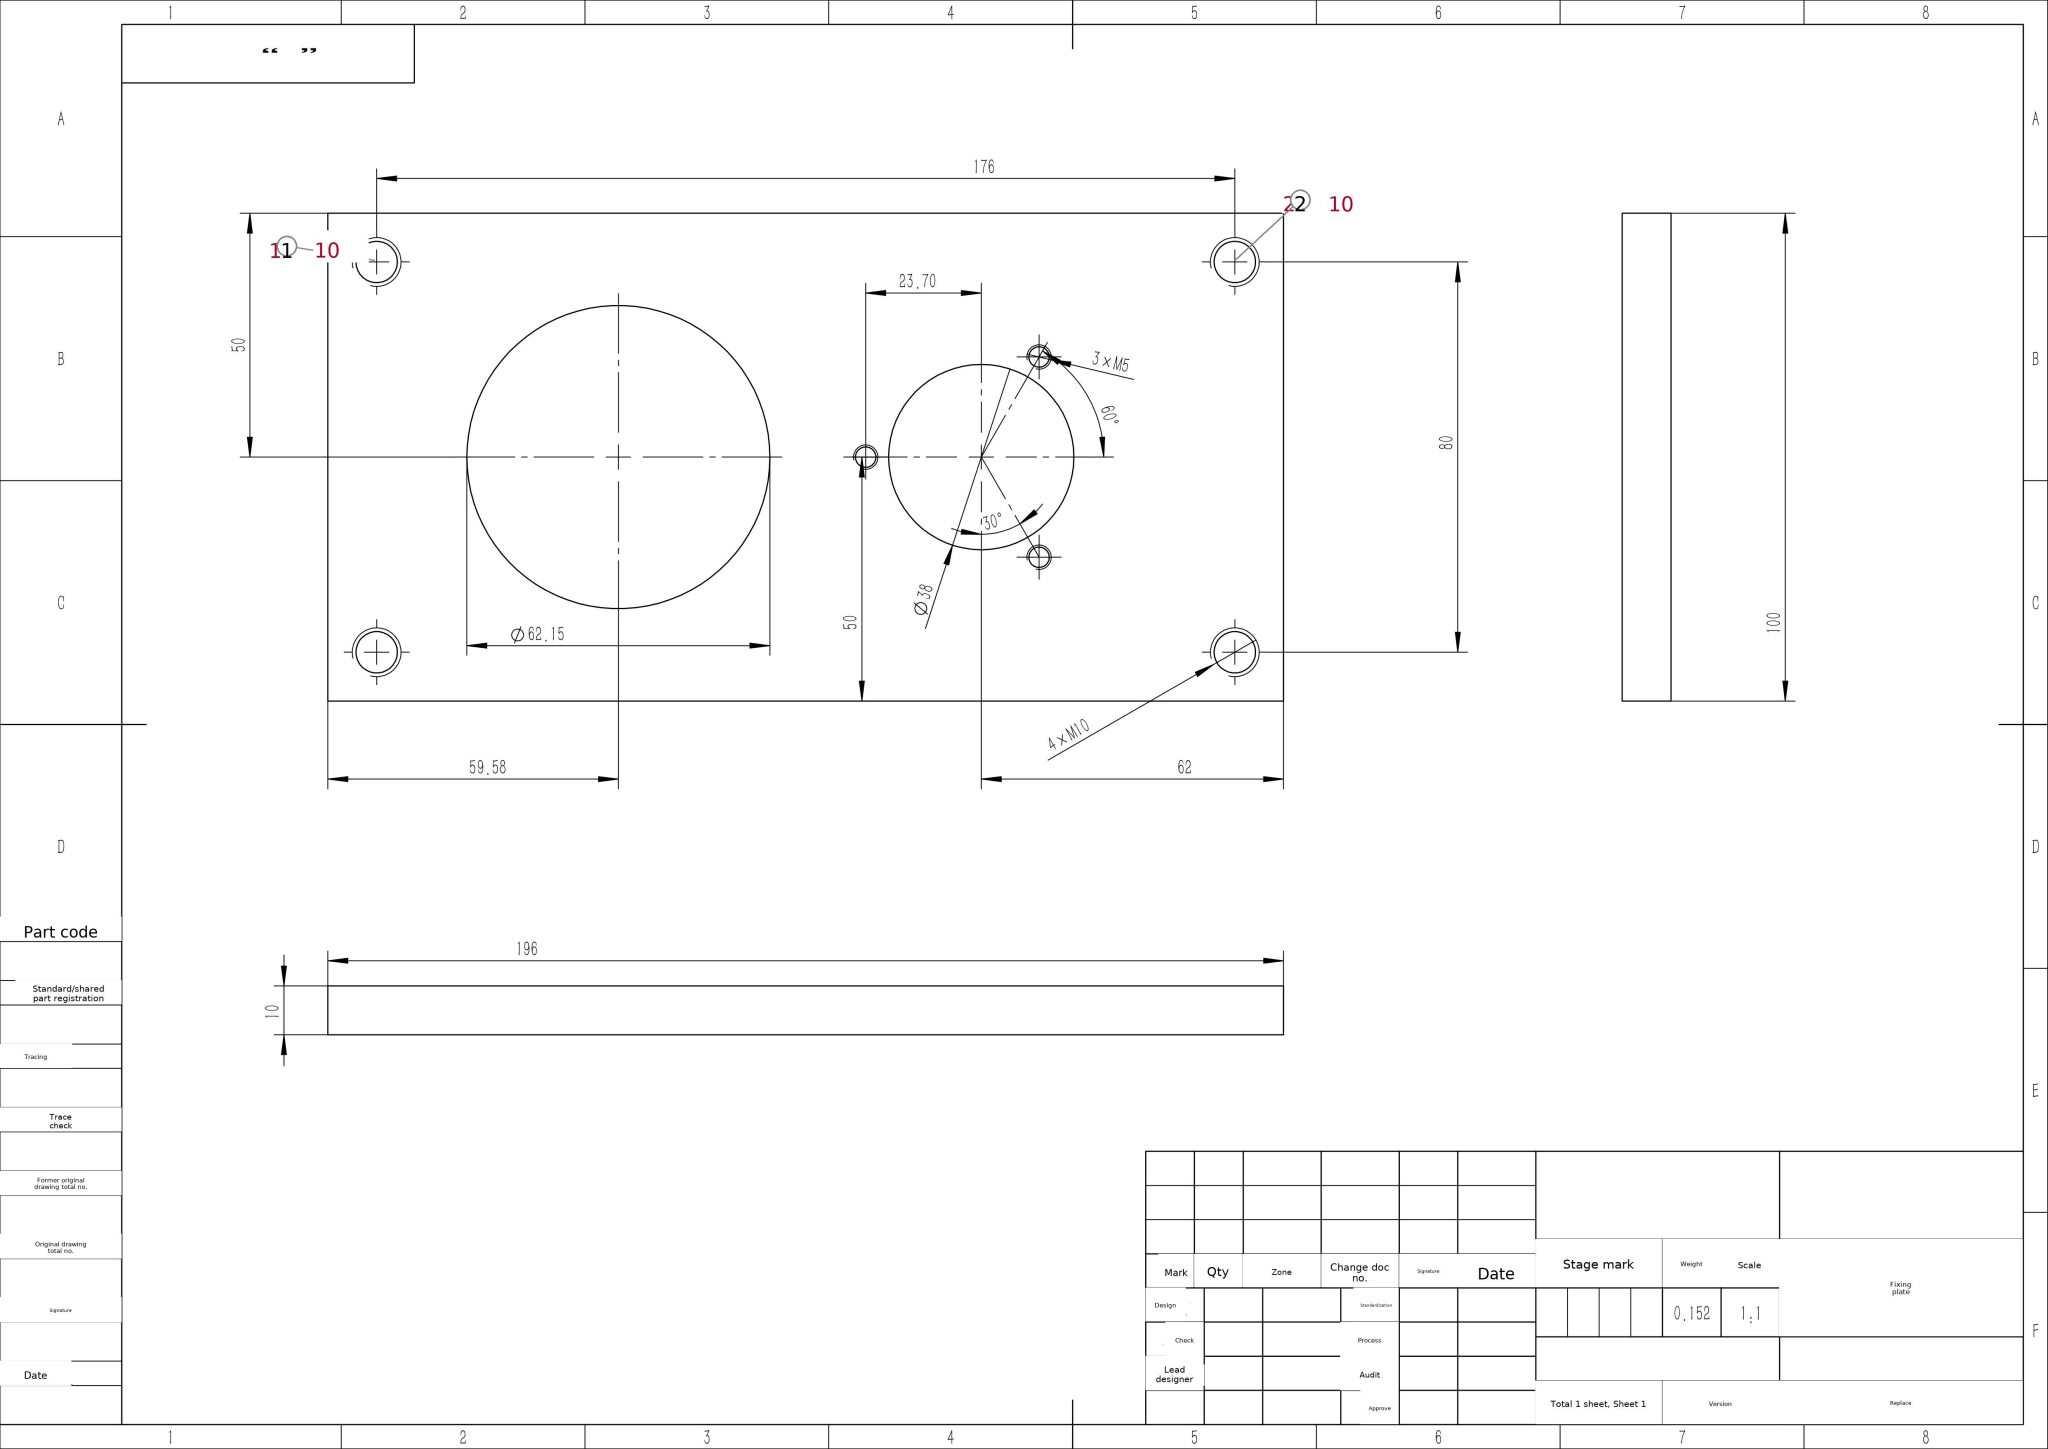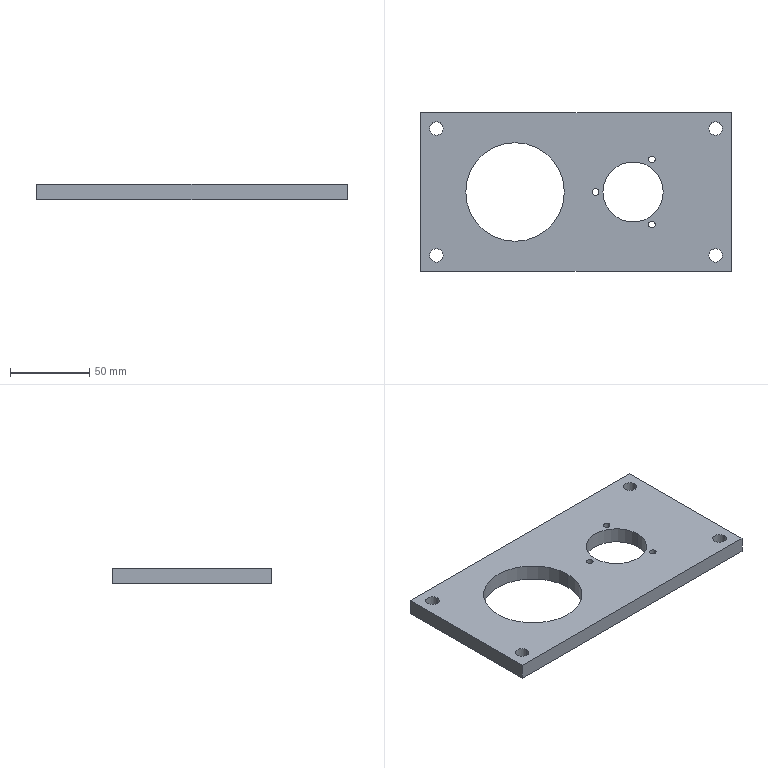Part | SolidWorks | mm | 1 solid | 24 faces | box 196 x 100 x 10 mm | volume 151636 mm3 | cylinder 18 | plane 6 | commonest cylinder face diameters 8.5 x8 4.2 x6 62.15 x2 38 x2
build123d program:
from build123d import *

# Parameters (mm, degrees)
SKETCH1_W           = 196
SKETCH1_H           = 100
BOSS_EXTRUDE1_DEPTH = 10
SKETCH2_R           = 31.075
SKETCH2_R_2         = 19
CUT_EXTRUDE1_DEPTH  = 10
M10_TAPPED_HOLE1_D  = 8.5
M5_TAPPED_HOLE1_D   = 4.2


with BuildPart() as part:
    # Sketch1 → Boss-Extrude1 (new body)
    with BuildSketch(Plane.XY):
        Rectangle(SKETCH1_W, SKETCH1_H)
    extrude(amount=BOSS_EXTRUDE1_DEPTH)

    # Sketch2 → Cut-Extrude1 (cut)
    with BuildSketch(Plane.XY):
        with Locations((-38.425, 0)):
            Circle(SKETCH2_R)
        with Locations((36, 0)):
            Circle(SKETCH2_R_2)
    extrude(amount=CUT_EXTRUDE1_DEPTH, mode=Mode.SUBTRACT)

    # M10 Tapped Hole1 (through all)
    with Locations(Plane.XY.offset(10)):
        with Locations((88, 40), (88, -40), (-88, -40), (-88, 40)):
            Hole(M10_TAPPED_HOLE1_D / 2)

    # M5 Tapped Hole1 (through all)
    with Locations(Plane.XY.offset(10)):
        with Locations((47.85, 20.525), (12.3, 0), (47.85, -20.525)):
            Hole(M5_TAPPED_HOLE1_D / 2)


solid = part.part
STEP:
#1=CARTESIAN_POINT('',(45.75,20.525,0.));
#2=VERTEX_POINT('',#1);
#3=CARTESIAN_POINT('',(49.95,20.525,0.));
#4=VERTEX_POINT('',#3);
#5=CARTESIAN_POINT('',(47.85,20.525,0.));
#6=DIRECTION('',(0.,0.,1.));
#7=DIRECTION('',(1.,0.,0.));
#8=AXIS2_PLACEMENT_3D('',#5,#6,#7);
#9=CIRCLE('',#8,2.1);
#10=EDGE_CURVE('',#2,#4,#9,.T.);
#11=ORIENTED_EDGE('',*,*,#10,.F.);
#12=CARTESIAN_POINT('',(45.75,20.525,10.));
#13=VERTEX_POINT('',#12);
#14=CARTESIAN_POINT('',(45.75,20.525,10.));
#15=DIRECTION('',(0.,0.,1.));
#16=VECTOR('',#15,1000.);
#17=LINE('',#14,#16);
#18=EDGE_CURVE('',#2,#13,#17,.T.);
#19=ORIENTED_EDGE('',*,*,#18,.T.);
#20=CARTESIAN_POINT('',(49.95,20.525,10.));
#21=VERTEX_POINT('',#20);
#22=CARTESIAN_POINT('',(47.85,20.525,10.));
#23=DIRECTION('',(0.,0.,1.));
#24=DIRECTION('',(1.,0.,0.));
#25=AXIS2_PLACEMENT_3D('',#22,#23,#24);
#26=CIRCLE('',#25,2.1);
#27=EDGE_CURVE('',#13,#21,#26,.T.);
#28=ORIENTED_EDGE('',*,*,#27,.T.);
#29=CARTESIAN_POINT('',(49.95,20.525,10.));
#30=DIRECTION('',(0.,0.,1.));
#31=VECTOR('',#30,1000.);
#32=LINE('',#29,#31);
#33=EDGE_CURVE('',#4,#21,#32,.T.);
#34=ORIENTED_EDGE('',*,*,#33,.F.);
#35=EDGE_LOOP('',(#11,#19,#28,#34));
#36=FACE_OUTER_BOUND('',#35,.T.);
#37=CARTESIAN_POINT('',(47.85,20.525,10.));
#38=DIRECTION('',(0.,0.,1.));
#39=DIRECTION('',(1.,0.,0.));
#40=AXIS2_PLACEMENT_3D('',#37,#38,#39);
#41=CYLINDRICAL_SURFACE('',#40,2.1);
#42=ADVANCED_FACE('',(#36),#41,.F.);
#43=CARTESIAN_POINT('',(10.2,-0.,0.));
#44=VERTEX_POINT('',#43);
#45=CARTESIAN_POINT('',(14.4,-0.,0.));
#46=VERTEX_POINT('',#45);
#47=CARTESIAN_POINT('',(12.3,-0.,0.));
#48=DIRECTION('',(0.,0.,1.));
#49=DIRECTION('',(1.,0.,0.));
#50=AXIS2_PLACEMENT_3D('',#47,#48,#49);
#51=CIRCLE('',#50,2.1);
#52=EDGE_CURVE('',#44,#46,#51,.T.);
#53=ORIENTED_EDGE('',*,*,#52,.F.);
#54=CARTESIAN_POINT('',(10.2,-0.,10.));
#55=VERTEX_POINT('',#54);
#56=CARTESIAN_POINT('',(10.2,-0.,10.));
#57=DIRECTION('',(0.,0.,1.));
#58=VECTOR('',#57,1000.);
#59=LINE('',#56,#58);
#60=EDGE_CURVE('',#44,#55,#59,.T.);
#61=ORIENTED_EDGE('',*,*,#60,.T.);
#62=CARTESIAN_POINT('',(14.4,-0.,10.));
#63=VERTEX_POINT('',#62);
#64=CARTESIAN_POINT('',(12.3,-0.,10.));
#65=DIRECTION('',(0.,0.,1.));
#66=DIRECTION('',(1.,0.,0.));
#67=AXIS2_PLACEMENT_3D('',#64,#65,#66);
#68=CIRCLE('',#67,2.1);
#69=EDGE_CURVE('',#55,#63,#68,.T.);
#70=ORIENTED_EDGE('',*,*,#69,.T.);
#71=CARTESIAN_POINT('',(14.4,-0.,10.));
#72=DIRECTION('',(0.,0.,1.));
#73=VECTOR('',#72,1000.);
#74=LINE('',#71,#73);
#75=EDGE_CURVE('',#46,#63,#74,.T.);
#76=ORIENTED_EDGE('',*,*,#75,.F.);
#77=EDGE_LOOP('',(#53,#61,#70,#76));
#78=FACE_OUTER_BOUND('',#77,.T.);
#79=CARTESIAN_POINT('',(12.3,-0.,10.));
#80=DIRECTION('',(0.,0.,1.));
#81=DIRECTION('',(1.,0.,0.));
#82=AXIS2_PLACEMENT_3D('',#79,#80,#81);
#83=CYLINDRICAL_SURFACE('',#82,2.1);
#84=ADVANCED_FACE('',(#78),#83,.F.);
#85=CARTESIAN_POINT('',(45.75,-20.525,0.));
#86=VERTEX_POINT('',#85);
#87=CARTESIAN_POINT('',(49.95,-20.525,0.));
#88=VERTEX_POINT('',#87);
#89=CARTESIAN_POINT('',(47.85,-20.525,0.));
#90=DIRECTION('',(0.,0.,1.));
#91=DIRECTION('',(1.,0.,0.));
#92=AXIS2_PLACEMENT_3D('',#89,#90,#91);
#93=CIRCLE('',#92,2.1);
#94=EDGE_CURVE('',#86,#88,#93,.T.);
#95=ORIENTED_EDGE('',*,*,#94,.F.);
#96=CARTESIAN_POINT('',(45.75,-20.525,10.));
#97=VERTEX_POINT('',#96);
#98=CARTESIAN_POINT('',(45.75,-20.525,10.));
#99=DIRECTION('',(0.,0.,1.));
#100=VECTOR('',#99,1000.);
#101=LINE('',#98,#100);
#102=EDGE_CURVE('',#86,#97,#101,.T.);
#103=ORIENTED_EDGE('',*,*,#102,.T.);
#104=CARTESIAN_POINT('',(49.95,-20.525,10.));
#105=VERTEX_POINT('',#104);
#106=CARTESIAN_POINT('',(47.85,-20.525,10.));
#107=DIRECTION('',(0.,0.,1.));
#108=DIRECTION('',(1.,0.,0.));
#109=AXIS2_PLACEMENT_3D('',#106,#107,#108);
#110=CIRCLE('',#109,2.1);
#111=EDGE_CURVE('',#97,#105,#110,.T.);
#112=ORIENTED_EDGE('',*,*,#111,.T.);
#113=CARTESIAN_POINT('',(49.95,-20.525,10.));
#114=DIRECTION('',(0.,0.,1.));
#115=VECTOR('',#114,1000.);
#116=LINE('',#113,#115);
#117=EDGE_CURVE('',#88,#105,#116,.T.);
#118=ORIENTED_EDGE('',*,*,#117,.F.);
#119=EDGE_LOOP('',(#95,#103,#112,#118));
#120=FACE_OUTER_BOUND('',#119,.T.);
#121=CARTESIAN_POINT('',(47.85,-20.525,10.));
#122=DIRECTION('',(0.,0.,1.));
#123=DIRECTION('',(1.,0.,0.));
#124=AXIS2_PLACEMENT_3D('',#121,#122,#123);
#125=CYLINDRICAL_SURFACE('',#124,2.1);
#126=ADVANCED_FACE('',(#120),#125,.F.);
#127=CARTESIAN_POINT('',(83.75,40.,0.));
#128=VERTEX_POINT('',#127);
#129=CARTESIAN_POINT('',(92.25,40.,0.));
#130=VERTEX_POINT('',#129);
#131=CARTESIAN_POINT('',(88.,40.,0.));
#132=DIRECTION('',(0.,0.,1.));
#133=DIRECTION('',(1.,0.,0.));
#134=AXIS2_PLACEMENT_3D('',#131,#132,#133);
#135=CIRCLE('',#134,4.25);
#136=EDGE_CURVE('',#128,#130,#135,.T.);
#137=ORIENTED_EDGE('',*,*,#136,.F.);
#138=CARTESIAN_POINT('',(83.75,40.,10.));
#139=VERTEX_POINT('',#138);
#140=CARTESIAN_POINT('',(83.75,40.,10.));
#141=DIRECTION('',(0.,0.,1.));
#142=VECTOR('',#141,1000.);
#143=LINE('',#140,#142);
#144=EDGE_CURVE('',#128,#139,#143,.T.);
#145=ORIENTED_EDGE('',*,*,#144,.T.);
#146=CARTESIAN_POINT('',(92.25,40.,10.));
#147=VERTEX_POINT('',#146);
#148=CARTESIAN_POINT('',(88.,40.,10.));
#149=DIRECTION('',(0.,0.,1.));
#150=DIRECTION('',(1.,0.,0.));
#151=AXIS2_PLACEMENT_3D('',#148,#149,#150);
#152=CIRCLE('',#151,4.25);
#153=EDGE_CURVE('',#139,#147,#152,.T.);
#154=ORIENTED_EDGE('',*,*,#153,.T.);
#155=CARTESIAN_POINT('',(92.25,40.,10.));
#156=DIRECTION('',(0.,0.,1.));
#157=VECTOR('',#156,1000.);
#158=LINE('',#155,#157);
#159=EDGE_CURVE('',#130,#147,#158,.T.);
#160=ORIENTED_EDGE('',*,*,#159,.F.);
#161=EDGE_LOOP('',(#137,#145,#154,#160));
#162=FACE_OUTER_BOUND('',#161,.T.);
#163=CARTESIAN_POINT('',(88.,40.,10.));
#164=DIRECTION('',(0.,0.,1.));
#165=DIRECTION('',(1.,0.,0.));
#166=AXIS2_PLACEMENT_3D('',#163,#164,#165);
#167=CYLINDRICAL_SURFACE('',#166,4.25);
#168=ADVANCED_FACE('',(#162),#167,.F.);
#169=CARTESIAN_POINT('',(83.75,-40.,0.));
#170=VERTEX_POINT('',#169);
#171=CARTESIAN_POINT('',(92.25,-40.,0.));
#172=VERTEX_POINT('',#171);
#173=CARTESIAN_POINT('',(88.,-40.,0.));
#174=DIRECTION('',(0.,0.,1.));
#175=DIRECTION('',(1.,0.,0.));
#176=AXIS2_PLACEMENT_3D('',#173,#174,#175);
#177=CIRCLE('',#176,4.25);
#178=EDGE_CURVE('',#170,#172,#177,.T.);
#179=ORIENTED_EDGE('',*,*,#178,.F.);
#180=CARTESIAN_POINT('',(83.75,-40.,10.));
#181=VERTEX_POINT('',#180);
#182=CARTESIAN_POINT('',(83.75,-40.,10.));
#183=DIRECTION('',(0.,0.,1.));
#184=VECTOR('',#183,1000.);
#185=LINE('',#182,#184);
#186=EDGE_CURVE('',#170,#181,#185,.T.);
#187=ORIENTED_EDGE('',*,*,#186,.T.);
#188=CARTESIAN_POINT('',(92.25,-40.,10.));
#189=VERTEX_POINT('',#188);
#190=CARTESIAN_POINT('',(88.,-40.,10.));
#191=DIRECTION('',(0.,0.,1.));
#192=DIRECTION('',(1.,0.,0.));
#193=AXIS2_PLACEMENT_3D('',#190,#191,#192);
#194=CIRCLE('',#193,4.25);
#195=EDGE_CURVE('',#181,#189,#194,.T.);
#196=ORIENTED_EDGE('',*,*,#195,.T.);
#197=CARTESIAN_POINT('',(92.25,-40.,10.));
#198=DIRECTION('',(0.,0.,1.));
#199=VECTOR('',#198,1000.);
#200=LINE('',#197,#199);
#201=EDGE_CURVE('',#172,#189,#200,.T.);
#202=ORIENTED_EDGE('',*,*,#201,.F.);
#203=EDGE_LOOP('',(#179,#187,#196,#202));
#204=FACE_OUTER_BOUND('',#203,.T.);
#205=CARTESIAN_POINT('',(88.,-40.,10.));
#206=DIRECTION('',(0.,0.,1.));
#207=DIRECTION('',(1.,0.,0.));
#208=AXIS2_PLACEMENT_3D('',#205,#206,#207);
#209=CYLINDRICAL_SURFACE('',#208,4.25);
#210=ADVANCED_FACE('',(#204),#209,.F.);
#211=CARTESIAN_POINT('',(-92.25,-40.,0.));
#212=VERTEX_POINT('',#211);
#213=CARTESIAN_POINT('',(-83.75,-40.,0.));
#214=VERTEX_POINT('',#213);
#215=CARTESIAN_POINT('',(-88.,-40.,0.));
#216=DIRECTION('',(0.,0.,1.));
#217=DIRECTION('',(1.,0.,0.));
#218=AXIS2_PLACEMENT_3D('',#215,#216,#217);
#219=CIRCLE('',#218,4.25);
#220=EDGE_CURVE('',#212,#214,#219,.T.);
#221=ORIENTED_EDGE('',*,*,#220,.F.);
#222=CARTESIAN_POINT('',(-92.25,-40.,10.));
#223=VERTEX_POINT('',#222);
#224=CARTESIAN_POINT('',(-92.25,-40.,10.));
#225=DIRECTION('',(0.,0.,1.));
#226=VECTOR('',#225,1000.);
#227=LINE('',#224,#226);
#228=EDGE_CURVE('',#212,#223,#227,.T.);
#229=ORIENTED_EDGE('',*,*,#228,.T.);
#230=CARTESIAN_POINT('',(-83.75,-40.,10.));
#231=VERTEX_POINT('',#230);
#232=CARTESIAN_POINT('',(-88.,-40.,10.));
#233=DIRECTION('',(0.,0.,1.));
#234=DIRECTION('',(1.,0.,0.));
#235=AXIS2_PLACEMENT_3D('',#232,#233,#234);
#236=CIRCLE('',#235,4.25);
#237=EDGE_CURVE('',#223,#231,#236,.T.);
#238=ORIENTED_EDGE('',*,*,#237,.T.);
#239=CARTESIAN_POINT('',(-83.75,-40.,10.));
#240=DIRECTION('',(0.,0.,1.));
#241=VECTOR('',#240,1000.);
#242=LINE('',#239,#241);
#243=EDGE_CURVE('',#214,#231,#242,.T.);
#244=ORIENTED_EDGE('',*,*,#243,.F.);
#245=EDGE_LOOP('',(#221,#229,#238,#244));
#246=FACE_OUTER_BOUND('',#245,.T.);
#247=CARTESIAN_POINT('',(-88.,-40.,10.));
#248=DIRECTION('',(0.,0.,1.));
#249=DIRECTION('',(1.,0.,0.));
#250=AXIS2_PLACEMENT_3D('',#247,#248,#249);
#251=CYLINDRICAL_SURFACE('',#250,4.25);
#252=ADVANCED_FACE('',(#246),#251,.F.);
#253=CARTESIAN_POINT('',(-92.25,40.,0.));
#254=VERTEX_POINT('',#253);
#255=CARTESIAN_POINT('',(-83.75,40.,0.));
#256=VERTEX_POINT('',#255);
#257=CARTESIAN_POINT('',(-88.,40.,0.));
#258=DIRECTION('',(0.,0.,1.));
#259=DIRECTION('',(1.,0.,0.));
#260=AXIS2_PLACEMENT_3D('',#257,#258,#259);
#261=CIRCLE('',#260,4.25);
#262=EDGE_CURVE('',#254,#256,#261,.T.);
#263=ORIENTED_EDGE('',*,*,#262,.F.);
#264=CARTESIAN_POINT('',(-92.25,40.,10.));
#265=VERTEX_POINT('',#264);
#266=CARTESIAN_POINT('',(-92.25,40.,10.));
#267=DIRECTION('',(0.,0.,1.));
#268=VECTOR('',#267,1000.);
#269=LINE('',#266,#268);
#270=EDGE_CURVE('',#254,#265,#269,.T.);
#271=ORIENTED_EDGE('',*,*,#270,.T.);
#272=CARTESIAN_POINT('',(-83.75,40.,10.));
#273=VERTEX_POINT('',#272);
#274=CARTESIAN_POINT('',(-88.,40.,10.));
#275=DIRECTION('',(0.,0.,1.));
#276=DIRECTION('',(1.,0.,0.));
#277=AXIS2_PLACEMENT_3D('',#274,#275,#276);
#278=CIRCLE('',#277,4.25);
#279=EDGE_CURVE('',#265,#273,#278,.T.);
#280=ORIENTED_EDGE('',*,*,#279,.T.);
#281=CARTESIAN_POINT('',(-83.75,40.,10.));
#282=DIRECTION('',(0.,0.,1.));
#283=VECTOR('',#282,1000.);
#284=LINE('',#281,#283);
#285=EDGE_CURVE('',#256,#273,#284,.T.);
#286=ORIENTED_EDGE('',*,*,#285,.F.);
#287=EDGE_LOOP('',(#263,#271,#280,#286));
#288=FACE_OUTER_BOUND('',#287,.T.);
#289=CARTESIAN_POINT('',(-88.,40.,10.));
#290=DIRECTION('',(0.,0.,1.));
#291=DIRECTION('',(1.,0.,0.));
#292=AXIS2_PLACEMENT_3D('',#289,#290,#291);
#293=CYLINDRICAL_SURFACE('',#292,4.25);
#294=ADVANCED_FACE('',(#288),#293,.F.);
#295=CARTESIAN_POINT('',(-69.5,0.,10.));
#296=VERTEX_POINT('',#295);
#297=CARTESIAN_POINT('',(-7.35,0.,10.));
#298=VERTEX_POINT('',#297);
#299=CARTESIAN_POINT('',(-38.425,0.,10.));
#300=DIRECTION('',(0.,0.,1.));
#301=DIRECTION('',(1.,0.,0.));
#302=AXIS2_PLACEMENT_3D('',#299,#300,#301);
#303=CIRCLE('',#302,31.075);
#304=EDGE_CURVE('',#296,#298,#303,.T.);
#305=ORIENTED_EDGE('',*,*,#304,.T.);
#306=CARTESIAN_POINT('',(-7.35,0.,0.));
#307=VERTEX_POINT('',#306);
#308=CARTESIAN_POINT('',(-7.35,0.,10.));
#309=DIRECTION('',(0.,0.,-1.));
#310=VECTOR('',#309,1000.);
#311=LINE('',#308,#310);
#312=EDGE_CURVE('',#298,#307,#311,.T.);
#313=ORIENTED_EDGE('',*,*,#312,.T.);
#314=CARTESIAN_POINT('',(-69.5,0.,0.));
#315=VERTEX_POINT('',#314);
#316=CARTESIAN_POINT('',(-38.425,0.,0.));
#317=DIRECTION('',(0.,0.,1.));
#318=DIRECTION('',(1.,0.,0.));
#319=AXIS2_PLACEMENT_3D('',#316,#317,#318);
#320=CIRCLE('',#319,31.075);
#321=EDGE_CURVE('',#315,#307,#320,.T.);
#322=ORIENTED_EDGE('',*,*,#321,.F.);
#323=CARTESIAN_POINT('',(-69.5,0.,10.));
#324=DIRECTION('',(0.,0.,-1.));
#325=VECTOR('',#324,1000.);
#326=LINE('',#323,#325);
#327=EDGE_CURVE('',#296,#315,#326,.T.);
#328=ORIENTED_EDGE('',*,*,#327,.F.);
#329=EDGE_LOOP('',(#305,#313,#322,#328));
#330=FACE_OUTER_BOUND('',#329,.T.);
#331=CARTESIAN_POINT('',(-38.425,0.,10.));
#332=DIRECTION('',(0.,0.,-1.));
#333=DIRECTION('',(-1.,0.,0.));
#334=AXIS2_PLACEMENT_3D('',#331,#332,#333);
#335=CYLINDRICAL_SURFACE('',#334,31.075);
#336=ADVANCED_FACE('',(#330),#335,.F.);
#337=CARTESIAN_POINT('',(17.,0.,10.));
#338=VERTEX_POINT('',#337);
#339=CARTESIAN_POINT('',(55.,0.,10.));
#340=VERTEX_POINT('',#339);
#341=CARTESIAN_POINT('',(36.,0.,10.));
#342=DIRECTION('',(0.,0.,1.));
#343=DIRECTION('',(1.,0.,0.));
#344=AXIS2_PLACEMENT_3D('',#341,#342,#343);
#345=CIRCLE('',#344,19.);
#346=EDGE_CURVE('',#338,#340,#345,.T.);
#347=ORIENTED_EDGE('',*,*,#346,.T.);
#348=CARTESIAN_POINT('',(55.,0.,0.));
#349=VERTEX_POINT('',#348);
#350=CARTESIAN_POINT('',(55.,0.,10.));
#351=DIRECTION('',(0.,0.,-1.));
#352=VECTOR('',#351,1000.);
#353=LINE('',#350,#352);
#354=EDGE_CURVE('',#340,#349,#353,.T.);
#355=ORIENTED_EDGE('',*,*,#354,.T.);
#356=CARTESIAN_POINT('',(17.,0.,0.));
#357=VERTEX_POINT('',#356);
#358=CARTESIAN_POINT('',(36.,0.,0.));
#359=DIRECTION('',(0.,0.,1.));
#360=DIRECTION('',(1.,0.,0.));
#361=AXIS2_PLACEMENT_3D('',#358,#359,#360);
#362=CIRCLE('',#361,19.);
#363=EDGE_CURVE('',#357,#349,#362,.T.);
#364=ORIENTED_EDGE('',*,*,#363,.F.);
#365=CARTESIAN_POINT('',(17.,0.,10.));
#366=DIRECTION('',(0.,0.,-1.));
#367=VECTOR('',#366,1000.);
#368=LINE('',#365,#367);
#369=EDGE_CURVE('',#338,#357,#368,.T.);
#370=ORIENTED_EDGE('',*,*,#369,.F.);
#371=EDGE_LOOP('',(#347,#355,#364,#370));
#372=FACE_OUTER_BOUND('',#371,.T.);
#373=CARTESIAN_POINT('',(36.,0.,10.));
#374=DIRECTION('',(0.,0.,-1.));
#375=DIRECTION('',(-1.,0.,0.));
#376=AXIS2_PLACEMENT_3D('',#373,#374,#375);
#377=CYLINDRICAL_SURFACE('',#376,19.);
#378=ADVANCED_FACE('',(#372),#377,.F.);
#379=CARTESIAN_POINT('',(98.,-50.,0.));
#380=VERTEX_POINT('',#379);
#381=CARTESIAN_POINT('',(98.,50.,0.));
#382=VERTEX_POINT('',#381);
#383=CARTESIAN_POINT('',(98.,50.,0.));
#384=DIRECTION('',(-0.,1.,0.));
#385=VECTOR('',#384,1000.);
#386=LINE('',#383,#385);
#387=EDGE_CURVE('',#380,#382,#386,.T.);
#388=ORIENTED_EDGE('',*,*,#387,.T.);
#389=CARTESIAN_POINT('',(98.,50.,10.));
#390=VERTEX_POINT('',#389);
#391=CARTESIAN_POINT('',(98.,50.,10.));
#392=DIRECTION('',(0.,0.,-1.));
#393=VECTOR('',#392,1000.);
#394=LINE('',#391,#393);
#395=EDGE_CURVE('',#390,#382,#394,.T.);
#396=ORIENTED_EDGE('',*,*,#395,.F.);
#397=CARTESIAN_POINT('',(98.,-50.,10.));
#398=VERTEX_POINT('',#397);
#399=CARTESIAN_POINT('',(98.,50.,10.));
#400=DIRECTION('',(-0.,1.,0.));
#401=VECTOR('',#400,1000.);
#402=LINE('',#399,#401);
#403=EDGE_CURVE('',#398,#390,#402,.T.);
#404=ORIENTED_EDGE('',*,*,#403,.F.);
#405=CARTESIAN_POINT('',(98.,-50.,10.));
#406=DIRECTION('',(0.,0.,-1.));
#407=VECTOR('',#406,1000.);
#408=LINE('',#405,#407);
#409=EDGE_CURVE('',#398,#380,#408,.T.);
#410=ORIENTED_EDGE('',*,*,#409,.T.);
#411=EDGE_LOOP('',(#388,#396,#404,#410));
#412=FACE_OUTER_BOUND('',#411,.T.);
#413=CARTESIAN_POINT('',(98.,50.,10.));
#414=DIRECTION('',(-1.,-0.,0.));
#415=DIRECTION('',(0.,-1.,0.));
#416=AXIS2_PLACEMENT_3D('',#413,#414,#415);
#417=PLANE('',#416);
#418=ADVANCED_FACE('',(#412),#417,.F.);
#419=CARTESIAN_POINT('',(-98.,50.,0.));
#420=VERTEX_POINT('',#419);
#421=CARTESIAN_POINT('',(-98.,50.,0.));
#422=DIRECTION('',(-1.,0.,0.));
#423=VECTOR('',#422,1000.);
#424=LINE('',#421,#423);
#425=EDGE_CURVE('',#382,#420,#424,.T.);
#426=ORIENTED_EDGE('',*,*,#425,.T.);
#427=CARTESIAN_POINT('',(-98.,50.,10.));
#428=VERTEX_POINT('',#427);
#429=CARTESIAN_POINT('',(-98.,50.,10.));
#430=DIRECTION('',(0.,0.,-1.));
#431=VECTOR('',#430,1000.);
#432=LINE('',#429,#431);
#433=EDGE_CURVE('',#428,#420,#432,.T.);
#434=ORIENTED_EDGE('',*,*,#433,.F.);
#435=CARTESIAN_POINT('',(-98.,50.,10.));
#436=DIRECTION('',(-1.,0.,0.));
#437=VECTOR('',#436,1000.);
#438=LINE('',#435,#437);
#439=EDGE_CURVE('',#390,#428,#438,.T.);
#440=ORIENTED_EDGE('',*,*,#439,.F.);
#441=ORIENTED_EDGE('',*,*,#395,.T.);
#442=EDGE_LOOP('',(#426,#434,#440,#441));
#443=FACE_OUTER_BOUND('',#442,.T.);
#444=CARTESIAN_POINT('',(-98.,50.,10.));
#445=DIRECTION('',(0.,-1.,0.));
#446=DIRECTION('',(0.,0.,-1.));
#447=AXIS2_PLACEMENT_3D('',#444,#445,#446);
#448=PLANE('',#447);
#449=ADVANCED_FACE('',(#443),#448,.F.);
#450=CARTESIAN_POINT('',(-98.,-50.,0.));
#451=VERTEX_POINT('',#450);
#452=CARTESIAN_POINT('',(-98.,50.,0.));
#453=DIRECTION('',(0.,-1.,0.));
#454=VECTOR('',#453,1000.);
#455=LINE('',#452,#454);
#456=EDGE_CURVE('',#420,#451,#455,.T.);
#457=ORIENTED_EDGE('',*,*,#456,.T.);
#458=CARTESIAN_POINT('',(-98.,-50.,10.));
#459=VERTEX_POINT('',#458);
#460=CARTESIAN_POINT('',(-98.,-50.,10.));
#461=DIRECTION('',(0.,0.,-1.));
#462=VECTOR('',#461,1000.);
#463=LINE('',#460,#462);
#464=EDGE_CURVE('',#459,#451,#463,.T.);
#465=ORIENTED_EDGE('',*,*,#464,.F.);
#466=CARTESIAN_POINT('',(-98.,50.,10.));
#467=DIRECTION('',(0.,-1.,0.));
#468=VECTOR('',#467,1000.);
#469=LINE('',#466,#468);
#470=EDGE_CURVE('',#428,#459,#469,.T.);
#471=ORIENTED_EDGE('',*,*,#470,.F.);
#472=ORIENTED_EDGE('',*,*,#433,.T.);
#473=EDGE_LOOP('',(#457,#465,#471,#472));
#474=FACE_OUTER_BOUND('',#473,.T.);
#475=CARTESIAN_POINT('',(-98.,50.,10.));
#476=DIRECTION('',(1.,0.,0.));
#477=DIRECTION('',(-0.,1.,0.));
#478=AXIS2_PLACEMENT_3D('',#475,#476,#477);
#479=PLANE('',#478);
#480=ADVANCED_FACE('',(#474),#479,.F.);
#481=CARTESIAN_POINT('',(-98.,-50.,0.));
#482=DIRECTION('',(1.,0.,0.));
#483=VECTOR('',#482,1000.);
#484=LINE('',#481,#483);
#485=EDGE_CURVE('',#451,#380,#484,.T.);
#486=ORIENTED_EDGE('',*,*,#485,.T.);
#487=ORIENTED_EDGE('',*,*,#409,.F.);
#488=CARTESIAN_POINT('',(-98.,-50.,10.));
#489=DIRECTION('',(1.,0.,0.));
#490=VECTOR('',#489,1000.);
#491=LINE('',#488,#490);
#492=EDGE_CURVE('',#459,#398,#491,.T.);
#493=ORIENTED_EDGE('',*,*,#492,.F.);
#494=ORIENTED_EDGE('',*,*,#464,.T.);
#495=EDGE_LOOP('',(#486,#487,#493,#494));
#496=FACE_OUTER_BOUND('',#495,.T.);
#497=CARTESIAN_POINT('',(-98.,-50.,10.));
#498=DIRECTION('',(0.,1.,0.));
#499=DIRECTION('',(0.,0.,1.));
#500=AXIS2_PLACEMENT_3D('',#497,#498,#499);
#501=PLANE('',#500);
#502=ADVANCED_FACE('',(#496),#501,.F.);
#503=CARTESIAN_POINT('',(47.85,20.525,10.));
#504=DIRECTION('',(0.,0.,1.));
#505=DIRECTION('',(1.,0.,0.));
#506=AXIS2_PLACEMENT_3D('',#503,#504,#505);
#507=CIRCLE('',#506,2.1);
#508=EDGE_CURVE('',#21,#13,#507,.T.);
#509=ORIENTED_EDGE('',*,*,#508,.F.);
#510=ORIENTED_EDGE('',*,*,#27,.F.);
#511=EDGE_LOOP('',(#509,#510));
#512=FACE_BOUND('',#511,.T.);
#513=CARTESIAN_POINT('',(12.3,-0.,10.));
#514=DIRECTION('',(0.,0.,1.));
#515=DIRECTION('',(1.,0.,0.));
#516=AXIS2_PLACEMENT_3D('',#513,#514,#515);
#517=CIRCLE('',#516,2.1);
#518=EDGE_CURVE('',#63,#55,#517,.T.);
#519=ORIENTED_EDGE('',*,*,#518,.F.);
#520=ORIENTED_EDGE('',*,*,#69,.F.);
#521=EDGE_LOOP('',(#519,#520));
#522=FACE_BOUND('',#521,.T.);
#523=CARTESIAN_POINT('',(47.85,-20.525,10.));
#524=DIRECTION('',(0.,0.,1.));
#525=DIRECTION('',(1.,0.,0.));
#526=AXIS2_PLACEMENT_3D('',#523,#524,#525);
#527=CIRCLE('',#526,2.1);
#528=EDGE_CURVE('',#105,#97,#527,.T.);
#529=ORIENTED_EDGE('',*,*,#528,.F.);
#530=ORIENTED_EDGE('',*,*,#111,.F.);
#531=EDGE_LOOP('',(#529,#530));
#532=FACE_BOUND('',#531,.T.);
#533=CARTESIAN_POINT('',(88.,40.,10.));
#534=DIRECTION('',(0.,0.,1.));
#535=DIRECTION('',(1.,0.,0.));
#536=AXIS2_PLACEMENT_3D('',#533,#534,#535);
#537=CIRCLE('',#536,4.25);
#538=EDGE_CURVE('',#147,#139,#537,.T.);
#539=ORIENTED_EDGE('',*,*,#538,.F.);
#540=ORIENTED_EDGE('',*,*,#153,.F.);
#541=EDGE_LOOP('',(#539,#540));
#542=FACE_BOUND('',#541,.T.);
#543=CARTESIAN_POINT('',(88.,-40.,10.));
#544=DIRECTION('',(0.,0.,1.));
#545=DIRECTION('',(1.,0.,0.));
#546=AXIS2_PLACEMENT_3D('',#543,#544,#545);
#547=CIRCLE('',#546,4.25);
#548=EDGE_CURVE('',#189,#181,#547,.T.);
#549=ORIENTED_EDGE('',*,*,#548,.F.);
#550=ORIENTED_EDGE('',*,*,#195,.F.);
#551=EDGE_LOOP('',(#549,#550));
#552=FACE_BOUND('',#551,.T.);
#553=CARTESIAN_POINT('',(-88.,-40.,10.));
#554=DIRECTION('',(0.,0.,1.));
#555=DIRECTION('',(1.,0.,0.));
#556=AXIS2_PLACEMENT_3D('',#553,#554,#555);
#557=CIRCLE('',#556,4.25);
#558=EDGE_CURVE('',#231,#223,#557,.T.);
#559=ORIENTED_EDGE('',*,*,#558,.F.);
#560=ORIENTED_EDGE('',*,*,#237,.F.);
#561=EDGE_LOOP('',(#559,#560));
#562=FACE_BOUND('',#561,.T.);
#563=CARTESIAN_POINT('',(-88.,40.,10.));
#564=DIRECTION('',(0.,0.,1.));
#565=DIRECTION('',(1.,0.,0.));
#566=AXIS2_PLACEMENT_3D('',#563,#564,#565);
#567=CIRCLE('',#566,4.25);
#568=EDGE_CURVE('',#273,#265,#567,.T.);
#569=ORIENTED_EDGE('',*,*,#568,.F.);
#570=ORIENTED_EDGE('',*,*,#279,.F.);
#571=EDGE_LOOP('',(#569,#570));
#572=FACE_BOUND('',#571,.T.);
#573=ORIENTED_EDGE('',*,*,#304,.F.);
#574=CARTESIAN_POINT('',(-38.425,0.,10.));
#575=DIRECTION('',(0.,0.,1.));
#576=DIRECTION('',(1.,0.,0.));
#577=AXIS2_PLACEMENT_3D('',#574,#575,#576);
#578=CIRCLE('',#577,31.075);
#579=EDGE_CURVE('',#298,#296,#578,.T.);
#580=ORIENTED_EDGE('',*,*,#579,.F.);
#581=EDGE_LOOP('',(#573,#580));
#582=FACE_BOUND('',#581,.T.);
#583=ORIENTED_EDGE('',*,*,#346,.F.);
#584=CARTESIAN_POINT('',(36.,0.,10.));
#585=DIRECTION('',(0.,0.,1.));
#586=DIRECTION('',(1.,0.,0.));
#587=AXIS2_PLACEMENT_3D('',#584,#585,#586);
#588=CIRCLE('',#587,19.);
#589=EDGE_CURVE('',#340,#338,#588,.T.);
#590=ORIENTED_EDGE('',*,*,#589,.F.);
#591=EDGE_LOOP('',(#583,#590));
#592=FACE_BOUND('',#591,.T.);
#593=ORIENTED_EDGE('',*,*,#403,.T.);
#594=ORIENTED_EDGE('',*,*,#439,.T.);
#595=ORIENTED_EDGE('',*,*,#470,.T.);
#596=ORIENTED_EDGE('',*,*,#492,.T.);
#597=EDGE_LOOP('',(#593,#594,#595,#596));
#598=FACE_OUTER_BOUND('',#597,.T.);
#599=CARTESIAN_POINT('',(0.,0.,10.));
#600=DIRECTION('',(0.,0.,1.));
#601=DIRECTION('',(1.,0.,0.));
#602=AXIS2_PLACEMENT_3D('',#599,#600,#601);
#603=PLANE('',#602);
#604=ADVANCED_FACE('',(#512,#522,#532,#542,#552,#562,#572,#582,#592,#598),#603,.T.);
#605=CARTESIAN_POINT('',(47.85,20.525,0.));
#606=DIRECTION('',(0.,0.,1.));
#607=DIRECTION('',(1.,0.,0.));
#608=AXIS2_PLACEMENT_3D('',#605,#606,#607);
#609=CIRCLE('',#608,2.1);
#610=EDGE_CURVE('',#4,#2,#609,.T.);
#611=ORIENTED_EDGE('',*,*,#610,.T.);
#612=ORIENTED_EDGE('',*,*,#10,.T.);
#613=EDGE_LOOP('',(#611,#612));
#614=FACE_BOUND('',#613,.T.);
#615=CARTESIAN_POINT('',(12.3,-0.,0.));
#616=DIRECTION('',(0.,0.,1.));
#617=DIRECTION('',(1.,0.,0.));
#618=AXIS2_PLACEMENT_3D('',#615,#616,#617);
#619=CIRCLE('',#618,2.1);
#620=EDGE_CURVE('',#46,#44,#619,.T.);
#621=ORIENTED_EDGE('',*,*,#620,.T.);
#622=ORIENTED_EDGE('',*,*,#52,.T.);
#623=EDGE_LOOP('',(#621,#622));
#624=FACE_BOUND('',#623,.T.);
#625=CARTESIAN_POINT('',(47.85,-20.525,0.));
#626=DIRECTION('',(0.,0.,1.));
#627=DIRECTION('',(1.,0.,0.));
#628=AXIS2_PLACEMENT_3D('',#625,#626,#627);
#629=CIRCLE('',#628,2.1);
#630=EDGE_CURVE('',#88,#86,#629,.T.);
#631=ORIENTED_EDGE('',*,*,#630,.T.);
#632=ORIENTED_EDGE('',*,*,#94,.T.);
#633=EDGE_LOOP('',(#631,#632));
#634=FACE_BOUND('',#633,.T.);
#635=CARTESIAN_POINT('',(88.,40.,0.));
#636=DIRECTION('',(0.,0.,1.));
#637=DIRECTION('',(1.,0.,0.));
#638=AXIS2_PLACEMENT_3D('',#635,#636,#637);
#639=CIRCLE('',#638,4.25);
#640=EDGE_CURVE('',#130,#128,#639,.T.);
#641=ORIENTED_EDGE('',*,*,#640,.T.);
#642=ORIENTED_EDGE('',*,*,#136,.T.);
#643=EDGE_LOOP('',(#641,#642));
#644=FACE_BOUND('',#643,.T.);
#645=CARTESIAN_POINT('',(88.,-40.,0.));
#646=DIRECTION('',(0.,0.,1.));
#647=DIRECTION('',(1.,0.,0.));
#648=AXIS2_PLACEMENT_3D('',#645,#646,#647);
#649=CIRCLE('',#648,4.25);
#650=EDGE_CURVE('',#172,#170,#649,.T.);
#651=ORIENTED_EDGE('',*,*,#650,.T.);
#652=ORIENTED_EDGE('',*,*,#178,.T.);
#653=EDGE_LOOP('',(#651,#652));
#654=FACE_BOUND('',#653,.T.);
#655=CARTESIAN_POINT('',(-88.,-40.,0.));
#656=DIRECTION('',(0.,0.,1.));
#657=DIRECTION('',(1.,0.,0.));
#658=AXIS2_PLACEMENT_3D('',#655,#656,#657);
#659=CIRCLE('',#658,4.25);
#660=EDGE_CURVE('',#214,#212,#659,.T.);
#661=ORIENTED_EDGE('',*,*,#660,.T.);
#662=ORIENTED_EDGE('',*,*,#220,.T.);
#663=EDGE_LOOP('',(#661,#662));
#664=FACE_BOUND('',#663,.T.);
#665=CARTESIAN_POINT('',(-88.,40.,0.));
#666=DIRECTION('',(0.,0.,1.));
#667=DIRECTION('',(1.,0.,0.));
#668=AXIS2_PLACEMENT_3D('',#665,#666,#667);
#669=CIRCLE('',#668,4.25);
#670=EDGE_CURVE('',#256,#254,#669,.T.);
#671=ORIENTED_EDGE('',*,*,#670,.T.);
#672=ORIENTED_EDGE('',*,*,#262,.T.);
#673=EDGE_LOOP('',(#671,#672));
#674=FACE_BOUND('',#673,.T.);
#675=ORIENTED_EDGE('',*,*,#321,.T.);
#676=CARTESIAN_POINT('',(-38.425,0.,0.));
#677=DIRECTION('',(0.,0.,1.));
#678=DIRECTION('',(1.,0.,0.));
#679=AXIS2_PLACEMENT_3D('',#676,#677,#678);
#680=CIRCLE('',#679,31.075);
#681=EDGE_CURVE('',#307,#315,#680,.T.);
#682=ORIENTED_EDGE('',*,*,#681,.T.);
#683=EDGE_LOOP('',(#675,#682));
#684=FACE_BOUND('',#683,.T.);
#685=ORIENTED_EDGE('',*,*,#363,.T.);
#686=CARTESIAN_POINT('',(36.,0.,0.));
#687=DIRECTION('',(0.,0.,1.));
#688=DIRECTION('',(1.,0.,0.));
#689=AXIS2_PLACEMENT_3D('',#686,#687,#688);
#690=CIRCLE('',#689,19.);
#691=EDGE_CURVE('',#349,#357,#690,.T.);
#692=ORIENTED_EDGE('',*,*,#691,.T.);
#693=EDGE_LOOP('',(#685,#692));
#694=FACE_BOUND('',#693,.T.);
#695=ORIENTED_EDGE('',*,*,#387,.F.);
#696=ORIENTED_EDGE('',*,*,#485,.F.);
#697=ORIENTED_EDGE('',*,*,#456,.F.);
#698=ORIENTED_EDGE('',*,*,#425,.F.);
#699=EDGE_LOOP('',(#695,#696,#697,#698));
#700=FACE_OUTER_BOUND('',#699,.T.);
#701=CARTESIAN_POINT('',(0.,0.,0.));
#702=DIRECTION('',(0.,0.,1.));
#703=DIRECTION('',(1.,0.,0.));
#704=AXIS2_PLACEMENT_3D('',#701,#702,#703);
#705=PLANE('',#704);
#706=ADVANCED_FACE('',(#614,#624,#634,#644,#654,#664,#674,#684,#694,#700),#705,.F.);
#707=ORIENTED_EDGE('',*,*,#354,.F.);
#708=ORIENTED_EDGE('',*,*,#589,.T.);
#709=ORIENTED_EDGE('',*,*,#369,.T.);
#710=ORIENTED_EDGE('',*,*,#691,.F.);
#711=EDGE_LOOP('',(#707,#708,#709,#710));
#712=FACE_OUTER_BOUND('',#711,.T.);
#713=CARTESIAN_POINT('',(36.,0.,10.));
#714=DIRECTION('',(0.,0.,-1.));
#715=DIRECTION('',(-1.,0.,0.));
#716=AXIS2_PLACEMENT_3D('',#713,#714,#715);
#717=CYLINDRICAL_SURFACE('',#716,19.);
#718=ADVANCED_FACE('',(#712),#717,.F.);
#719=ORIENTED_EDGE('',*,*,#312,.F.);
#720=ORIENTED_EDGE('',*,*,#579,.T.);
#721=ORIENTED_EDGE('',*,*,#327,.T.);
#722=ORIENTED_EDGE('',*,*,#681,.F.);
#723=EDGE_LOOP('',(#719,#720,#721,#722));
#724=FACE_OUTER_BOUND('',#723,.T.);
#725=CARTESIAN_POINT('',(-38.425,0.,10.));
#726=DIRECTION('',(0.,0.,-1.));
#727=DIRECTION('',(-1.,0.,0.));
#728=AXIS2_PLACEMENT_3D('',#725,#726,#727);
#729=CYLINDRICAL_SURFACE('',#728,31.075);
#730=ADVANCED_FACE('',(#724),#729,.F.);
#731=ORIENTED_EDGE('',*,*,#270,.F.);
#732=ORIENTED_EDGE('',*,*,#670,.F.);
#733=ORIENTED_EDGE('',*,*,#285,.T.);
#734=ORIENTED_EDGE('',*,*,#568,.T.);
#735=EDGE_LOOP('',(#731,#732,#733,#734));
#736=FACE_OUTER_BOUND('',#735,.T.);
#737=CARTESIAN_POINT('',(-88.,40.,10.));
#738=DIRECTION('',(0.,0.,1.));
#739=DIRECTION('',(1.,0.,0.));
#740=AXIS2_PLACEMENT_3D('',#737,#738,#739);
#741=CYLINDRICAL_SURFACE('',#740,4.25);
#742=ADVANCED_FACE('',(#736),#741,.F.);
#743=ORIENTED_EDGE('',*,*,#228,.F.);
#744=ORIENTED_EDGE('',*,*,#660,.F.);
#745=ORIENTED_EDGE('',*,*,#243,.T.);
#746=ORIENTED_EDGE('',*,*,#558,.T.);
#747=EDGE_LOOP('',(#743,#744,#745,#746));
#748=FACE_OUTER_BOUND('',#747,.T.);
#749=CARTESIAN_POINT('',(-88.,-40.,10.));
#750=DIRECTION('',(0.,0.,1.));
#751=DIRECTION('',(1.,0.,0.));
#752=AXIS2_PLACEMENT_3D('',#749,#750,#751);
#753=CYLINDRICAL_SURFACE('',#752,4.25);
#754=ADVANCED_FACE('',(#748),#753,.F.);
#755=ORIENTED_EDGE('',*,*,#186,.F.);
#756=ORIENTED_EDGE('',*,*,#650,.F.);
#757=ORIENTED_EDGE('',*,*,#201,.T.);
#758=ORIENTED_EDGE('',*,*,#548,.T.);
#759=EDGE_LOOP('',(#755,#756,#757,#758));
#760=FACE_OUTER_BOUND('',#759,.T.);
#761=CARTESIAN_POINT('',(88.,-40.,10.));
#762=DIRECTION('',(0.,0.,1.));
#763=DIRECTION('',(1.,0.,0.));
#764=AXIS2_PLACEMENT_3D('',#761,#762,#763);
#765=CYLINDRICAL_SURFACE('',#764,4.25);
#766=ADVANCED_FACE('',(#760),#765,.F.);
#767=ORIENTED_EDGE('',*,*,#144,.F.);
#768=ORIENTED_EDGE('',*,*,#640,.F.);
#769=ORIENTED_EDGE('',*,*,#159,.T.);
#770=ORIENTED_EDGE('',*,*,#538,.T.);
#771=EDGE_LOOP('',(#767,#768,#769,#770));
#772=FACE_OUTER_BOUND('',#771,.T.);
#773=CARTESIAN_POINT('',(88.,40.,10.));
#774=DIRECTION('',(0.,0.,1.));
#775=DIRECTION('',(1.,0.,0.));
#776=AXIS2_PLACEMENT_3D('',#773,#774,#775);
#777=CYLINDRICAL_SURFACE('',#776,4.25);
#778=ADVANCED_FACE('',(#772),#777,.F.);
#779=ORIENTED_EDGE('',*,*,#102,.F.);
#780=ORIENTED_EDGE('',*,*,#630,.F.);
#781=ORIENTED_EDGE('',*,*,#117,.T.);
#782=ORIENTED_EDGE('',*,*,#528,.T.);
#783=EDGE_LOOP('',(#779,#780,#781,#782));
#784=FACE_OUTER_BOUND('',#783,.T.);
#785=CARTESIAN_POINT('',(47.85,-20.525,10.));
#786=DIRECTION('',(0.,0.,1.));
#787=DIRECTION('',(1.,0.,0.));
#788=AXIS2_PLACEMENT_3D('',#785,#786,#787);
#789=CYLINDRICAL_SURFACE('',#788,2.1);
#790=ADVANCED_FACE('',(#784),#789,.F.);
#791=ORIENTED_EDGE('',*,*,#60,.F.);
#792=ORIENTED_EDGE('',*,*,#620,.F.);
#793=ORIENTED_EDGE('',*,*,#75,.T.);
#794=ORIENTED_EDGE('',*,*,#518,.T.);
#795=EDGE_LOOP('',(#791,#792,#793,#794));
#796=FACE_OUTER_BOUND('',#795,.T.);
#797=CARTESIAN_POINT('',(12.3,-0.,10.));
#798=DIRECTION('',(0.,0.,1.));
#799=DIRECTION('',(1.,0.,0.));
#800=AXIS2_PLACEMENT_3D('',#797,#798,#799);
#801=CYLINDRICAL_SURFACE('',#800,2.1);
#802=ADVANCED_FACE('',(#796),#801,.F.);
#803=ORIENTED_EDGE('',*,*,#18,.F.);
#804=ORIENTED_EDGE('',*,*,#610,.F.);
#805=ORIENTED_EDGE('',*,*,#33,.T.);
#806=ORIENTED_EDGE('',*,*,#508,.T.);
#807=EDGE_LOOP('',(#803,#804,#805,#806));
#808=FACE_OUTER_BOUND('',#807,.T.);
#809=CARTESIAN_POINT('',(47.85,20.525,10.));
#810=DIRECTION('',(0.,0.,1.));
#811=DIRECTION('',(1.,0.,0.));
#812=AXIS2_PLACEMENT_3D('',#809,#810,#811);
#813=CYLINDRICAL_SURFACE('',#812,2.1);
#814=ADVANCED_FACE('',(#808),#813,.F.);
#815=CLOSED_SHELL('',(#42,#84,#126,#168,#210,#252,#294,#336,#378,#418,#449,#480,#502,#604,#706,#718,#730,#742,#754,#766,#778,#790,#802,#814));
#816=MANIFOLD_SOLID_BREP('',#815);
#817=CARTESIAN_POINT('',(0.,0.,0.));
#818=DIRECTION('',(0.,0.,1.));
#819=DIRECTION('',(1.,0.,0.));
#820=AXIS2_PLACEMENT_3D('',#817,#818,#819);
#821=(LENGTH_UNIT()NAMED_UNIT(*)SI_UNIT(.MILLI.,.METRE.));
#822=UNCERTAINTY_MEASURE_WITH_UNIT(LENGTH_MEASURE(0.00001),#821,'','');
#823=(NAMED_UNIT(*)PLANE_ANGLE_UNIT()SI_UNIT($,.RADIAN.));
#824=(NAMED_UNIT(*)SI_UNIT($,.STERADIAN.)SOLID_ANGLE_UNIT());
#825=(GEOMETRIC_REPRESENTATION_CONTEXT(3)GLOBAL_UNCERTAINTY_ASSIGNED_CONTEXT((#822))GLOBAL_UNIT_ASSIGNED_CONTEXT((#821,#823,#824))REPRESENTATION_CONTEXT('',''));
#826=ADVANCED_BREP_SHAPE_REPRESENTATION('',(#816,#820),#825);